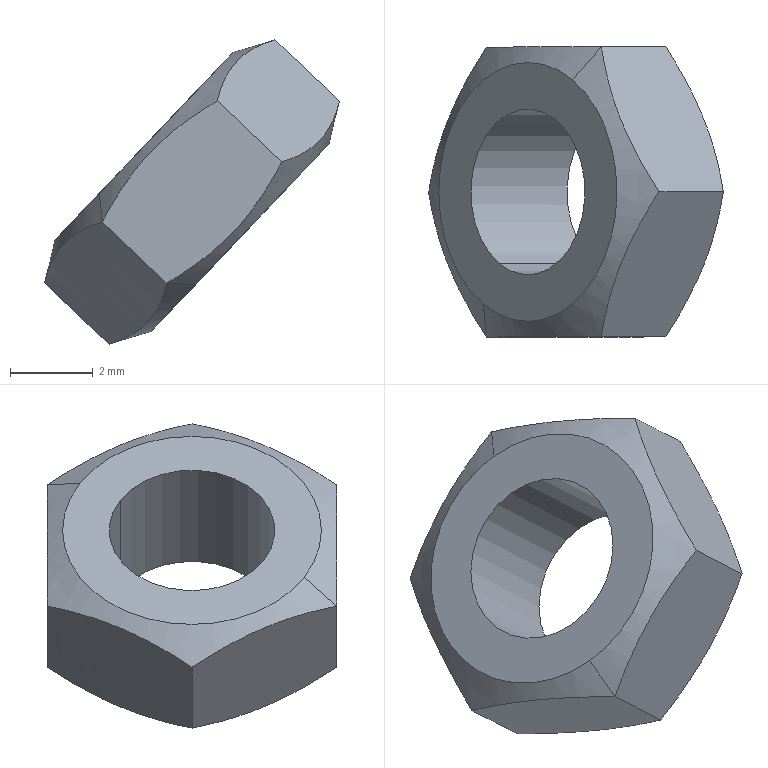Component | SolidWorks | 100-1_hex nuts, style 1-grades ab gb_GB_FASTENER_NUT_SNAB1 M4-N-1 | 1 solid | 14 faces | box 7.11 x 7 x 7.34 mm | volume 91 mm3 | plane 8 | cone 4 | cylinder 2 | commonest cylinder face diameters 4 x2
STEP:
#1=COLOUR_RGB('',0.7922,0.8196,0.9333);
#2=FILL_AREA_STYLE_COLOUR('',#1);
#3=FILL_AREA_STYLE('',(#2));
#4=SURFACE_STYLE_FILL_AREA(#3);
#5=SURFACE_SIDE_STYLE('',(#4));
#6=SURFACE_STYLE_USAGE(.BOTH.,#5);
#7=PRESENTATION_STYLE_ASSIGNMENT((#6));
#8=CARTESIAN_POINT('',(20.163,50.208,-80.248));
#9=VERTEX_POINT('',#8);
#10=CARTESIAN_POINT('',(20.248,50.422,-80.159));
#11=VERTEX_POINT('',#10);
#12=CARTESIAN_POINT('',(20.205,50.315,-80.204));
#13=DIRECTION('',(-0.7258,-0.,0.6879));
#14=DIRECTION('',(0.3439,0.866,0.3629));
#15=AXIS2_PLACEMENT_3D('',#12,#13,#14);
#16=CIRCLE('',#15,0.123);
#17=EDGE_CURVE('',#9,#11,#16,.T.);
#18=ORIENTED_EDGE('',*,*,#17,.T.);
#19=CARTESIAN_POINT('',(20.205,50.315,-80.204));
#20=DIRECTION('',(-0.7258,-0.,0.6879));
#21=DIRECTION('',(0.3439,0.866,0.3629));
#22=AXIS2_PLACEMENT_3D('',#19,#20,#21);
#23=CIRCLE('',#22,0.123);
#24=EDGE_CURVE('',#11,#9,#23,.T.);
#25=ORIENTED_EDGE('',*,*,#24,.T.);
#26=EDGE_LOOP('',(#18,#25));
#27=FACE_OUTER_BOUND('',#26,.T.);
#28=CARTESIAN_POINT('',(20.233,50.383,-80.175));
#29=VERTEX_POINT('',#28);
#30=CARTESIAN_POINT('',(20.178,50.247,-80.232));
#31=VERTEX_POINT('',#30);
#32=CARTESIAN_POINT('',(20.205,50.315,-80.204));
#33=DIRECTION('',(-0.7258,-0.,0.6879));
#34=DIRECTION('',(-0.3439,-0.866,-0.3629));
#35=AXIS2_PLACEMENT_3D('',#32,#33,#34);
#36=CIRCLE('',#35,0.07874);
#37=EDGE_CURVE('',#29,#31,#36,.T.);
#38=ORIENTED_EDGE('',*,*,#37,.F.);
#39=CARTESIAN_POINT('',(20.205,50.315,-80.204));
#40=DIRECTION('',(0.7258,0.,-0.6879));
#41=DIRECTION('',(-0.3439,-0.866,-0.3629));
#42=AXIS2_PLACEMENT_3D('',#39,#40,#41);
#43=CIRCLE('',#42,0.07874);
#44=EDGE_CURVE('',#29,#31,#43,.T.);
#45=ORIENTED_EDGE('',*,*,#44,.T.);
#46=EDGE_LOOP('',(#38,#45));
#47=FACE_BOUND('',#46,.T.);
#48=CARTESIAN_POINT('',(20.151,50.177,-80.262));
#49=DIRECTION('',(0.7258,0.,-0.6879));
#50=DIRECTION('',(-0.3439,-0.866,-0.3629));
#51=AXIS2_PLACEMENT_3D('',#48,#49,#50);
#52=PLANE('',#51);
#53=ADVANCED_FACE('',(#27,#47),#52,.F.);
#54=CARTESIAN_POINT('',(20.255,50.208,-80.335));
#55=VERTEX_POINT('',#54);
#56=CARTESIAN_POINT('',(20.227,50.177,-80.334));
#57=VERTEX_POINT('',#56);
#58=CARTESIAN_POINT('',(20.255,50.208,-80.335));
#59=DIRECTION('',(-0.6608,-0.75,0.02965));
#60=VECTOR('',#59,39.37);
#61=LINE('',#58,#60);
#62=EDGE_CURVE('',#55,#57,#61,.T.);
#63=ORIENTED_EDGE('',*,*,#62,.F.);
#64=CARTESIAN_POINT('',(20.339,50.422,-80.246));
#65=VERTEX_POINT('',#64);
#66=CARTESIAN_POINT('',(20.297,50.315,-80.29));
#67=DIRECTION('',(-0.7258,-0.,0.6879));
#68=DIRECTION('',(0.3439,0.866,0.3629));
#69=AXIS2_PLACEMENT_3D('',#66,#67,#68);
#70=CIRCLE('',#69,0.123);
#71=EDGE_CURVE('',#55,#65,#70,.T.);
#72=ORIENTED_EDGE('',*,*,#71,.T.);
#73=CARTESIAN_POINT('',(20.336,50.453,-80.218));
#74=VERTEX_POINT('',#73);
#75=CARTESIAN_POINT('',(20.339,50.422,-80.246));
#76=DIRECTION('',(-0.06505,0.75,0.6582));
#77=VECTOR('',#76,39.37);
#78=LINE('',#75,#77);
#79=EDGE_CURVE('',#65,#74,#78,.T.);
#80=ORIENTED_EDGE('',*,*,#79,.T.);
#81=CARTESIAN_POINT('',(20.391,50.315,-80.161));
#82=VERTEX_POINT('',#81);
#83=CARTESIAN_POINT('',(20.336,50.453,-80.218));
#84=CARTESIAN_POINT('',(20.34,50.447,-80.217));
#85=CARTESIAN_POINT('',(20.344,50.441,-80.216));
#86=CARTESIAN_POINT('',(20.349,50.433,-80.214));
#87=CARTESIAN_POINT('',(20.35,50.43,-80.213));
#88=CARTESIAN_POINT('',(20.353,50.426,-80.212));
#89=CARTESIAN_POINT('',(20.354,50.424,-80.212));
#90=CARTESIAN_POINT('',(20.355,50.422,-80.211));
#91=CARTESIAN_POINT('',(20.356,50.42,-80.211));
#92=CARTESIAN_POINT('',(20.356,50.419,-80.21));
#93=CARTESIAN_POINT('',(20.36,50.413,-80.209));
#94=CARTESIAN_POINT('',(20.363,50.407,-80.207));
#95=CARTESIAN_POINT('',(20.368,50.396,-80.203));
#96=CARTESIAN_POINT('',(20.37,50.39,-80.2));
#97=CARTESIAN_POINT('',(20.375,50.378,-80.196));
#98=CARTESIAN_POINT('',(20.377,50.372,-80.193));
#99=CARTESIAN_POINT('',(20.38,50.364,-80.189));
#100=CARTESIAN_POINT('',(20.381,50.361,-80.187));
#101=CARTESIAN_POINT('',(20.382,50.356,-80.185));
#102=CARTESIAN_POINT('',(20.383,50.354,-80.184));
#103=CARTESIAN_POINT('',(20.383,50.352,-80.183));
#104=CARTESIAN_POINT('',(20.384,50.351,-80.182));
#105=CARTESIAN_POINT('',(20.384,50.35,-80.181));
#106=CARTESIAN_POINT('',(20.387,50.338,-80.175));
#107=CARTESIAN_POINT('',(20.389,50.327,-80.168));
#108=CARTESIAN_POINT('',(20.391,50.315,-80.161));
#109=B_SPLINE_CURVE_WITH_KNOTS('',3,(#83,#84,#85,#86,#87,#88,#89,#90,#91,#92,#93,#94,#95,#96,#97,#98,#99,#100,#101,#102,#103,#104,#105,#106,#107,#108),.UNSPECIFIED.,.F.,.F.,(4,2,2,1,2,2,2,2,2,2,1,2,2,4),(0.,0.125,0.1875,0.2187,0.2344,0.25,0.375,0.5,0.625,0.6875,0.7188,0.7344,0.75,1.),.UNSPECIFIED.);
#110=EDGE_CURVE('',#74,#82,#109,.T.);
#111=ORIENTED_EDGE('',*,*,#110,.T.);
#112=CARTESIAN_POINT('',(20.336,50.177,-80.218));
#113=VERTEX_POINT('',#112);
#114=CARTESIAN_POINT('',(20.391,50.315,-80.161));
#115=CARTESIAN_POINT('',(20.39,50.309,-80.164));
#116=CARTESIAN_POINT('',(20.389,50.303,-80.168));
#117=CARTESIAN_POINT('',(20.388,50.295,-80.173));
#118=CARTESIAN_POINT('',(20.387,50.292,-80.175));
#119=CARTESIAN_POINT('',(20.386,50.288,-80.177));
#120=CARTESIAN_POINT('',(20.385,50.286,-80.178));
#121=CARTESIAN_POINT('',(20.385,50.284,-80.18));
#122=CARTESIAN_POINT('',(20.385,50.282,-80.18));
#123=CARTESIAN_POINT('',(20.384,50.282,-80.181));
#124=CARTESIAN_POINT('',(20.381,50.269,-80.188));
#125=CARTESIAN_POINT('',(20.377,50.258,-80.193));
#126=CARTESIAN_POINT('',(20.372,50.243,-80.199));
#127=CARTESIAN_POINT('',(20.37,50.24,-80.2));
#128=CARTESIAN_POINT('',(20.368,50.234,-80.203));
#129=CARTESIAN_POINT('',(20.367,50.231,-80.204));
#130=CARTESIAN_POINT('',(20.364,50.226,-80.206));
#131=CARTESIAN_POINT('',(20.362,50.223,-80.207));
#132=CARTESIAN_POINT('',(20.36,50.218,-80.208));
#133=CARTESIAN_POINT('',(20.36,50.217,-80.209));
#134=CARTESIAN_POINT('',(20.358,50.214,-80.209));
#135=CARTESIAN_POINT('',(20.357,50.212,-80.21));
#136=CARTESIAN_POINT('',(20.351,50.2,-80.214));
#137=CARTESIAN_POINT('',(20.344,50.189,-80.216));
#138=CARTESIAN_POINT('',(20.336,50.177,-80.218));
#139=B_SPLINE_CURVE_WITH_KNOTS('',3,(#114,#115,#116,#117,#118,#119,#120,#121,#122,#123,#124,#125,#126,#127,#128,#129,#130,#131,#132,#133,#134,#135,#136,#137,#138),.UNSPECIFIED.,.F.,.F.,(4,2,2,1,2,2,2,2,2,2,2,2,4),(0.,0.125,0.1875,0.2188,0.2344,0.25,0.5,0.5625,0.625,0.6875,0.7188,0.75,1.),.UNSPECIFIED.);
#140=EDGE_CURVE('',#82,#113,#139,.T.);
#141=ORIENTED_EDGE('',*,*,#140,.T.);
#142=CARTESIAN_POINT('',(20.336,50.177,-80.218));
#143=CARTESIAN_POINT('',(20.333,50.177,-80.225));
#144=CARTESIAN_POINT('',(20.33,50.177,-80.231));
#145=CARTESIAN_POINT('',(20.325,50.177,-80.239));
#146=CARTESIAN_POINT('',(20.323,50.177,-80.242));
#147=CARTESIAN_POINT('',(20.32,50.177,-80.246));
#148=CARTESIAN_POINT('',(20.319,50.177,-80.248));
#149=CARTESIAN_POINT('',(20.318,50.177,-80.25));
#150=CARTESIAN_POINT('',(20.317,50.177,-80.252));
#151=CARTESIAN_POINT('',(20.316,50.177,-80.252));
#152=CARTESIAN_POINT('',(20.312,50.177,-80.259));
#153=CARTESIAN_POINT('',(20.308,50.177,-80.264));
#154=CARTESIAN_POINT('',(20.3,50.177,-80.275));
#155=CARTESIAN_POINT('',(20.295,50.177,-80.28));
#156=CARTESIAN_POINT('',(20.286,50.177,-80.289));
#157=CARTESIAN_POINT('',(20.281,50.177,-80.294));
#158=CARTESIAN_POINT('',(20.274,50.177,-80.301));
#159=CARTESIAN_POINT('',(20.271,50.177,-80.303));
#160=CARTESIAN_POINT('',(20.267,50.177,-80.306));
#161=CARTESIAN_POINT('',(20.265,50.177,-80.308));
#162=CARTESIAN_POINT('',(20.263,50.177,-80.309));
#163=CARTESIAN_POINT('',(20.262,50.177,-80.31));
#164=CARTESIAN_POINT('',(20.261,50.177,-80.311));
#165=CARTESIAN_POINT('',(20.25,50.177,-80.319));
#166=CARTESIAN_POINT('',(20.239,50.177,-80.327));
#167=CARTESIAN_POINT('',(20.227,50.177,-80.334));
#168=B_SPLINE_CURVE_WITH_KNOTS('',3,(#142,#143,#144,#145,#146,#147,#148,#149,#150,#151,#152,#153,#154,#155,#156,#157,#158,#159,#160,#161,#162,#163,#164,#165,#166,#167),.UNSPECIFIED.,.F.,.F.,(4,2,2,1,2,2,2,2,2,2,1,2,2,4),(0.,0.125,0.1875,0.2188,0.2344,0.25,0.375,0.5,0.625,0.6875,0.7188,0.7344,0.75,1.),.UNSPECIFIED.);
#169=EDGE_CURVE('',#113,#57,#168,.T.);
#170=ORIENTED_EDGE('',*,*,#169,.T.);
#171=EDGE_LOOP('',(#63,#72,#80,#111,#141,#170));
#172=FACE_OUTER_BOUND('',#171,.T.);
#173=CARTESIAN_POINT('',(20.297,50.315,-80.29));
#174=DIRECTION('',(-0.7258,-0.,0.6879));
#175=DIRECTION('',(0.3439,0.866,0.3629));
#176=AXIS2_PLACEMENT_3D('',#173,#174,#175);
#177=CONICAL_SURFACE('',#176,0.123,1.047);
#178=ADVANCED_FACE('',(#172),#177,.T.);
#179=CARTESIAN_POINT('',(20.275,50.453,-80.16));
#180=VERTEX_POINT('',#179);
#181=CARTESIAN_POINT('',(20.275,50.453,-80.16));
#182=DIRECTION('',(0.6608,0.75,-0.02965));
#183=VECTOR('',#182,39.37);
#184=LINE('',#181,#183);
#185=EDGE_CURVE('',#11,#180,#184,.T.);
#186=ORIENTED_EDGE('',*,*,#185,.F.);
#187=ORIENTED_EDGE('',*,*,#17,.F.);
#188=CARTESIAN_POINT('',(20.166,50.177,-80.276));
#189=VERTEX_POINT('',#188);
#190=CARTESIAN_POINT('',(20.166,50.177,-80.276));
#191=DIRECTION('',(0.06505,-0.75,-0.6582));
#192=VECTOR('',#191,39.37);
#193=LINE('',#190,#192);
#194=EDGE_CURVE('',#9,#189,#193,.T.);
#195=ORIENTED_EDGE('',*,*,#194,.T.);
#196=CARTESIAN_POINT('',(20.275,50.177,-80.16));
#197=VERTEX_POINT('',#196);
#198=CARTESIAN_POINT('',(20.166,50.177,-80.276));
#199=CARTESIAN_POINT('',(20.169,50.177,-80.27));
#200=CARTESIAN_POINT('',(20.172,50.177,-80.264));
#201=CARTESIAN_POINT('',(20.177,50.177,-80.255));
#202=CARTESIAN_POINT('',(20.179,50.177,-80.252));
#203=CARTESIAN_POINT('',(20.182,50.177,-80.248));
#204=CARTESIAN_POINT('',(20.183,50.177,-80.246));
#205=CARTESIAN_POINT('',(20.185,50.177,-80.244));
#206=CARTESIAN_POINT('',(20.185,50.177,-80.242));
#207=CARTESIAN_POINT('',(20.186,50.177,-80.242));
#208=CARTESIAN_POINT('',(20.19,50.177,-80.235));
#209=CARTESIAN_POINT('',(20.194,50.177,-80.23));
#210=CARTESIAN_POINT('',(20.203,50.177,-80.22));
#211=CARTESIAN_POINT('',(20.207,50.177,-80.215));
#212=CARTESIAN_POINT('',(20.216,50.177,-80.205));
#213=CARTESIAN_POINT('',(20.221,50.177,-80.2));
#214=CARTESIAN_POINT('',(20.228,50.177,-80.194));
#215=CARTESIAN_POINT('',(20.231,50.177,-80.191));
#216=CARTESIAN_POINT('',(20.235,50.177,-80.188));
#217=CARTESIAN_POINT('',(20.237,50.177,-80.186));
#218=CARTESIAN_POINT('',(20.239,50.177,-80.185));
#219=CARTESIAN_POINT('',(20.24,50.177,-80.184));
#220=CARTESIAN_POINT('',(20.241,50.177,-80.183));
#221=CARTESIAN_POINT('',(20.252,50.177,-80.175));
#222=CARTESIAN_POINT('',(20.263,50.177,-80.168));
#223=CARTESIAN_POINT('',(20.275,50.177,-80.16));
#224=B_SPLINE_CURVE_WITH_KNOTS('',3,(#198,#199,#200,#201,#202,#203,#204,#205,#206,#207,#208,#209,#210,#211,#212,#213,#214,#215,#216,#217,#218,#219,#220,#221,#222,#223),.UNSPECIFIED.,.F.,.F.,(4,2,2,1,2,2,2,2,2,2,1,2,2,4),(0.,0.125,0.1875,0.2188,0.2344,0.25,0.375,0.5,0.625,0.6875,0.7188,0.7344,0.75,1.),.UNSPECIFIED.);
#225=EDGE_CURVE('',#189,#197,#224,.T.);
#226=ORIENTED_EDGE('',*,*,#225,.T.);
#227=CARTESIAN_POINT('',(20.33,50.315,-80.103));
#228=VERTEX_POINT('',#227);
#229=CARTESIAN_POINT('',(20.275,50.177,-80.16));
#230=CARTESIAN_POINT('',(20.276,50.183,-80.157));
#231=CARTESIAN_POINT('',(20.277,50.189,-80.153));
#232=CARTESIAN_POINT('',(20.279,50.197,-80.148));
#233=CARTESIAN_POINT('',(20.28,50.2,-80.146));
#234=CARTESIAN_POINT('',(20.281,50.204,-80.144));
#235=CARTESIAN_POINT('',(20.281,50.206,-80.143));
#236=CARTESIAN_POINT('',(20.282,50.208,-80.142));
#237=CARTESIAN_POINT('',(20.282,50.21,-80.141));
#238=CARTESIAN_POINT('',(20.283,50.214,-80.138));
#239=CARTESIAN_POINT('',(20.284,50.217,-80.137));
#240=CARTESIAN_POINT('',(20.286,50.223,-80.134));
#241=CARTESIAN_POINT('',(20.286,50.226,-80.132));
#242=CARTESIAN_POINT('',(20.289,50.234,-80.128));
#243=CARTESIAN_POINT('',(20.291,50.24,-80.125));
#244=CARTESIAN_POINT('',(20.296,50.252,-80.121));
#245=CARTESIAN_POINT('',(20.298,50.258,-80.118));
#246=CARTESIAN_POINT('',(20.302,50.266,-80.115));
#247=CARTESIAN_POINT('',(20.304,50.269,-80.114));
#248=CARTESIAN_POINT('',(20.306,50.273,-80.113));
#249=CARTESIAN_POINT('',(20.307,50.276,-80.112));
#250=CARTESIAN_POINT('',(20.308,50.278,-80.112));
#251=CARTESIAN_POINT('',(20.309,50.279,-80.111));
#252=CARTESIAN_POINT('',(20.31,50.28,-80.111));
#253=CARTESIAN_POINT('',(20.316,50.292,-80.107));
#254=CARTESIAN_POINT('',(20.322,50.303,-80.105));
#255=CARTESIAN_POINT('',(20.33,50.315,-80.103));
#256=B_SPLINE_CURVE_WITH_KNOTS('',3,(#229,#230,#231,#232,#233,#234,#235,#236,#237,#238,#239,#240,#241,#242,#243,#244,#245,#246,#247,#248,#249,#250,#251,#252,#253,#254,#255),.UNSPECIFIED.,.F.,.F.,(4,2,2,2,2,2,2,2,2,2,1,2,2,4),(0.,0.125,0.1875,0.2188,0.25,0.3125,0.375,0.5,0.625,0.6875,0.7188,0.7344,0.75,1.),.UNSPECIFIED.);
#257=EDGE_CURVE('',#197,#228,#256,.T.);
#258=ORIENTED_EDGE('',*,*,#257,.T.);
#259=CARTESIAN_POINT('',(20.33,50.315,-80.103));
#260=CARTESIAN_POINT('',(20.326,50.321,-80.104));
#261=CARTESIAN_POINT('',(20.323,50.327,-80.105));
#262=CARTESIAN_POINT('',(20.318,50.335,-80.107));
#263=CARTESIAN_POINT('',(20.316,50.338,-80.108));
#264=CARTESIAN_POINT('',(20.314,50.342,-80.109));
#265=CARTESIAN_POINT('',(20.313,50.344,-80.109));
#266=CARTESIAN_POINT('',(20.311,50.346,-80.11));
#267=CARTESIAN_POINT('',(20.311,50.348,-80.11));
#268=CARTESIAN_POINT('',(20.31,50.348,-80.11));
#269=CARTESIAN_POINT('',(20.307,50.355,-80.112));
#270=CARTESIAN_POINT('',(20.304,50.361,-80.114));
#271=CARTESIAN_POINT('',(20.299,50.372,-80.118));
#272=CARTESIAN_POINT('',(20.296,50.378,-80.121));
#273=CARTESIAN_POINT('',(20.291,50.39,-80.125));
#274=CARTESIAN_POINT('',(20.289,50.395,-80.128));
#275=CARTESIAN_POINT('',(20.286,50.404,-80.132));
#276=CARTESIAN_POINT('',(20.286,50.407,-80.134));
#277=CARTESIAN_POINT('',(20.284,50.411,-80.136));
#278=CARTESIAN_POINT('',(20.284,50.413,-80.137));
#279=CARTESIAN_POINT('',(20.283,50.416,-80.138));
#280=CARTESIAN_POINT('',(20.283,50.417,-80.139));
#281=CARTESIAN_POINT('',(20.282,50.418,-80.139));
#282=CARTESIAN_POINT('',(20.279,50.43,-80.146));
#283=CARTESIAN_POINT('',(20.277,50.441,-80.153));
#284=CARTESIAN_POINT('',(20.275,50.453,-80.16));
#285=B_SPLINE_CURVE_WITH_KNOTS('',3,(#259,#260,#261,#262,#263,#264,#265,#266,#267,#268,#269,#270,#271,#272,#273,#274,#275,#276,#277,#278,#279,#280,#281,#282,#283,#284),.UNSPECIFIED.,.F.,.F.,(4,2,2,1,2,2,2,2,2,2,1,2,2,4),(0.,0.125,0.1875,0.2188,0.2344,0.25,0.375,0.5,0.625,0.6875,0.7187,0.7344,0.75,1.),.UNSPECIFIED.);
#286=EDGE_CURVE('',#228,#180,#285,.T.);
#287=ORIENTED_EDGE('',*,*,#286,.T.);
#288=EDGE_LOOP('',(#186,#187,#195,#226,#258,#287));
#289=FACE_OUTER_BOUND('',#288,.T.);
#290=CARTESIAN_POINT('',(20.221,50.315,-80.218));
#291=DIRECTION('',(0.7258,0.,-0.6879));
#292=DIRECTION('',(-0.3439,-0.866,-0.3629));
#293=AXIS2_PLACEMENT_3D('',#290,#291,#292);
#294=CONICAL_SURFACE('',#293,0.1591,1.047);
#295=ADVANCED_FACE('',(#289),#294,.T.);
#296=CARTESIAN_POINT('',(20.324,50.383,-80.262));
#297=VERTEX_POINT('',#296);
#298=CARTESIAN_POINT('',(20.233,50.383,-80.175));
#299=DIRECTION('',(0.7258,0.,-0.6879));
#300=VECTOR('',#299,39.37);
#301=LINE('',#298,#300);
#302=EDGE_CURVE('',#29,#297,#301,.T.);
#303=ORIENTED_EDGE('',*,*,#302,.F.);
#304=ORIENTED_EDGE('',*,*,#37,.T.);
#305=CARTESIAN_POINT('',(20.27,50.247,-80.319));
#306=VERTEX_POINT('',#305);
#307=CARTESIAN_POINT('',(20.178,50.247,-80.232));
#308=DIRECTION('',(0.7258,0.,-0.6879));
#309=VECTOR('',#308,39.37);
#310=LINE('',#307,#309);
#311=EDGE_CURVE('',#31,#306,#310,.T.);
#312=ORIENTED_EDGE('',*,*,#311,.T.);
#313=CARTESIAN_POINT('',(20.297,50.315,-80.29));
#314=DIRECTION('',(0.7258,0.,-0.6879));
#315=DIRECTION('',(-0.3439,-0.866,-0.3629));
#316=AXIS2_PLACEMENT_3D('',#313,#314,#315);
#317=CIRCLE('',#316,0.07874);
#318=EDGE_CURVE('',#306,#297,#317,.T.);
#319=ORIENTED_EDGE('',*,*,#318,.T.);
#320=EDGE_LOOP('',(#303,#304,#312,#319));
#321=FACE_OUTER_BOUND('',#320,.T.);
#322=CARTESIAN_POINT('',(20.205,50.315,-80.204));
#323=DIRECTION('',(0.7258,0.,-0.6879));
#324=DIRECTION('',(-0.3439,-0.866,-0.3629));
#325=AXIS2_PLACEMENT_3D('',#322,#323,#324);
#326=CYLINDRICAL_SURFACE('',#325,0.07874);
#327=ADVANCED_FACE('',(#321),#326,.F.);
#328=CARTESIAN_POINT('',(20.297,50.315,-80.29));
#329=DIRECTION('',(-0.7258,-0.,0.6879));
#330=DIRECTION('',(-0.3439,-0.866,-0.3629));
#331=AXIS2_PLACEMENT_3D('',#328,#329,#330);
#332=CIRCLE('',#331,0.07874);
#333=EDGE_CURVE('',#306,#297,#332,.T.);
#334=ORIENTED_EDGE('',*,*,#333,.T.);
#335=ORIENTED_EDGE('',*,*,#318,.F.);
#336=EDGE_LOOP('',(#334,#335));
#337=FACE_BOUND('',#336,.T.);
#338=CARTESIAN_POINT('',(20.297,50.315,-80.29));
#339=DIRECTION('',(-0.7258,-0.,0.6879));
#340=DIRECTION('',(0.3439,0.866,0.3629));
#341=AXIS2_PLACEMENT_3D('',#338,#339,#340);
#342=CIRCLE('',#341,0.123);
#343=EDGE_CURVE('',#65,#55,#342,.T.);
#344=ORIENTED_EDGE('',*,*,#343,.F.);
#345=ORIENTED_EDGE('',*,*,#71,.F.);
#346=EDGE_LOOP('',(#344,#345));
#347=FACE_OUTER_BOUND('',#346,.T.);
#348=CARTESIAN_POINT('',(20.242,50.177,-80.348));
#349=DIRECTION('',(0.7258,0.,-0.6879));
#350=DIRECTION('',(-0.3439,-0.866,-0.3629));
#351=AXIS2_PLACEMENT_3D('',#348,#349,#350);
#352=PLANE('',#351);
#353=ADVANCED_FACE('',(#337,#347),#352,.T.);
#354=CARTESIAN_POINT('',(20.172,50.315,-80.392));
#355=VERTEX_POINT('',#354);
#356=CARTESIAN_POINT('',(20.227,50.177,-80.334));
#357=CARTESIAN_POINT('',(20.226,50.183,-80.338));
#358=CARTESIAN_POINT('',(20.225,50.189,-80.341));
#359=CARTESIAN_POINT('',(20.223,50.197,-80.346));
#360=CARTESIAN_POINT('',(20.223,50.2,-80.348));
#361=CARTESIAN_POINT('',(20.222,50.204,-80.35));
#362=CARTESIAN_POINT('',(20.221,50.206,-80.352));
#363=CARTESIAN_POINT('',(20.221,50.208,-80.353));
#364=CARTESIAN_POINT('',(20.22,50.21,-80.354));
#365=CARTESIAN_POINT('',(20.22,50.21,-80.354));
#366=CARTESIAN_POINT('',(20.218,50.217,-80.358));
#367=CARTESIAN_POINT('',(20.217,50.223,-80.361));
#368=CARTESIAN_POINT('',(20.213,50.234,-80.366));
#369=CARTESIAN_POINT('',(20.211,50.24,-80.369));
#370=CARTESIAN_POINT('',(20.206,50.252,-80.374));
#371=CARTESIAN_POINT('',(20.204,50.258,-80.376));
#372=CARTESIAN_POINT('',(20.2,50.266,-80.379));
#373=CARTESIAN_POINT('',(20.198,50.269,-80.38));
#374=CARTESIAN_POINT('',(20.196,50.273,-80.381));
#375=CARTESIAN_POINT('',(20.195,50.276,-80.382));
#376=CARTESIAN_POINT('',(20.194,50.278,-80.383));
#377=CARTESIAN_POINT('',(20.193,50.279,-80.383));
#378=CARTESIAN_POINT('',(20.193,50.28,-80.383));
#379=CARTESIAN_POINT('',(20.186,50.292,-80.387));
#380=CARTESIAN_POINT('',(20.18,50.303,-80.389));
#381=CARTESIAN_POINT('',(20.172,50.315,-80.392));
#382=B_SPLINE_CURVE_WITH_KNOTS('',3,(#356,#357,#358,#359,#360,#361,#362,#363,#364,#365,#366,#367,#368,#369,#370,#371,#372,#373,#374,#375,#376,#377,#378,#379,#380,#381),.UNSPECIFIED.,.F.,.F.,(4,2,2,1,2,2,2,2,2,2,1,2,2,4),(0.,0.125,0.1875,0.2187,0.2344,0.25,0.375,0.5,0.625,0.6875,0.7187,0.7344,0.75,1.),.UNSPECIFIED.);
#383=EDGE_CURVE('',#57,#355,#382,.T.);
#384=ORIENTED_EDGE('',*,*,#383,.F.);
#385=CARTESIAN_POINT('',(20.151,50.177,-80.262));
#386=DIRECTION('',(0.7258,0.,-0.6879));
#387=VECTOR('',#386,39.37);
#388=LINE('',#385,#387);
#389=EDGE_CURVE('',#189,#57,#388,.T.);
#390=ORIENTED_EDGE('',*,*,#389,.F.);
#391=CARTESIAN_POINT('',(20.111,50.315,-80.334));
#392=VERTEX_POINT('',#391);
#393=CARTESIAN_POINT('',(20.111,50.315,-80.334));
#394=CARTESIAN_POINT('',(20.112,50.309,-80.33));
#395=CARTESIAN_POINT('',(20.113,50.303,-80.326));
#396=CARTESIAN_POINT('',(20.115,50.295,-80.321));
#397=CARTESIAN_POINT('',(20.115,50.292,-80.319));
#398=CARTESIAN_POINT('',(20.116,50.288,-80.317));
#399=CARTESIAN_POINT('',(20.117,50.286,-80.316));
#400=CARTESIAN_POINT('',(20.117,50.284,-80.315));
#401=CARTESIAN_POINT('',(20.118,50.282,-80.314));
#402=CARTESIAN_POINT('',(20.118,50.282,-80.314));
#403=CARTESIAN_POINT('',(20.12,50.275,-80.31));
#404=CARTESIAN_POINT('',(20.121,50.269,-80.307));
#405=CARTESIAN_POINT('',(20.125,50.258,-80.301));
#406=CARTESIAN_POINT('',(20.127,50.252,-80.299));
#407=CARTESIAN_POINT('',(20.132,50.24,-80.294));
#408=CARTESIAN_POINT('',(20.134,50.235,-80.292));
#409=CARTESIAN_POINT('',(20.138,50.226,-80.289));
#410=CARTESIAN_POINT('',(20.14,50.223,-80.288));
#411=CARTESIAN_POINT('',(20.142,50.219,-80.286));
#412=CARTESIAN_POINT('',(20.143,50.216,-80.285));
#413=CARTESIAN_POINT('',(20.144,50.214,-80.285));
#414=CARTESIAN_POINT('',(20.145,50.213,-80.284));
#415=CARTESIAN_POINT('',(20.145,50.212,-80.284));
#416=CARTESIAN_POINT('',(20.152,50.2,-80.281));
#417=CARTESIAN_POINT('',(20.158,50.189,-80.278));
#418=CARTESIAN_POINT('',(20.166,50.177,-80.276));
#419=B_SPLINE_CURVE_WITH_KNOTS('',3,(#393,#394,#395,#396,#397,#398,#399,#400,#401,#402,#403,#404,#405,#406,#407,#408,#409,#410,#411,#412,#413,#414,#415,#416,#417,#418),.UNSPECIFIED.,.F.,.F.,(4,2,2,1,2,2,2,2,2,2,1,2,2,4),(0.,0.125,0.1875,0.2187,0.2344,0.25,0.375,0.5,0.625,0.6875,0.7187,0.7344,0.75,1.),.UNSPECIFIED.);
#420=EDGE_CURVE('',#392,#189,#419,.T.);
#421=ORIENTED_EDGE('',*,*,#420,.F.);
#422=CARTESIAN_POINT('',(20.096,50.315,-80.319));
#423=DIRECTION('',(0.7258,0.,-0.6879));
#424=VECTOR('',#423,39.37);
#425=LINE('',#422,#424);
#426=EDGE_CURVE('',#392,#355,#425,.T.);
#427=ORIENTED_EDGE('',*,*,#426,.T.);
#428=EDGE_LOOP('',(#384,#390,#421,#427));
#429=FACE_OUTER_BOUND('',#428,.T.);
#430=CARTESIAN_POINT('',(20.151,50.177,-80.262));
#431=DIRECTION('',(-0.5957,-0.5,-0.6286));
#432=DIRECTION('',(-0.7258,-0.,0.6879));
#433=AXIS2_PLACEMENT_3D('',#430,#431,#432);
#434=PLANE('',#433);
#435=ADVANCED_FACE('',(#429),#434,.T.);
#436=CARTESIAN_POINT('',(20.227,50.453,-80.334));
#437=VERTEX_POINT('',#436);
#438=CARTESIAN_POINT('',(20.172,50.315,-80.392));
#439=CARTESIAN_POINT('',(20.176,50.321,-80.39));
#440=CARTESIAN_POINT('',(20.18,50.327,-80.389));
#441=CARTESIAN_POINT('',(20.185,50.335,-80.387));
#442=CARTESIAN_POINT('',(20.186,50.338,-80.387));
#443=CARTESIAN_POINT('',(20.189,50.342,-80.385));
#444=CARTESIAN_POINT('',(20.189,50.343,-80.385));
#445=CARTESIAN_POINT('',(20.191,50.346,-80.384));
#446=CARTESIAN_POINT('',(20.192,50.347,-80.384));
#447=CARTESIAN_POINT('',(20.194,50.352,-80.383));
#448=CARTESIAN_POINT('',(20.195,50.355,-80.382));
#449=CARTESIAN_POINT('',(20.198,50.361,-80.38));
#450=CARTESIAN_POINT('',(20.2,50.363,-80.379));
#451=CARTESIAN_POINT('',(20.204,50.372,-80.376));
#452=CARTESIAN_POINT('',(20.206,50.378,-80.374));
#453=CARTESIAN_POINT('',(20.211,50.39,-80.369));
#454=CARTESIAN_POINT('',(20.213,50.395,-80.366));
#455=CARTESIAN_POINT('',(20.216,50.404,-80.362));
#456=CARTESIAN_POINT('',(20.217,50.407,-80.361));
#457=CARTESIAN_POINT('',(20.218,50.411,-80.358));
#458=CARTESIAN_POINT('',(20.219,50.413,-80.357));
#459=CARTESIAN_POINT('',(20.219,50.416,-80.356));
#460=CARTESIAN_POINT('',(20.22,50.417,-80.355));
#461=CARTESIAN_POINT('',(20.22,50.418,-80.355));
#462=CARTESIAN_POINT('',(20.223,50.43,-80.348));
#463=CARTESIAN_POINT('',(20.225,50.441,-80.341));
#464=CARTESIAN_POINT('',(20.227,50.453,-80.334));
#465=B_SPLINE_CURVE_WITH_KNOTS('',3,(#438,#439,#440,#441,#442,#443,#444,#445,#446,#447,#448,#449,#450,#451,#452,#453,#454,#455,#456,#457,#458,#459,#460,#461,#462,#463,#464),.UNSPECIFIED.,.F.,.F.,(4,2,2,2,2,2,2,2,2,2,1,2,2,4),(0.,0.125,0.1875,0.2188,0.25,0.3125,0.375,0.5,0.625,0.6875,0.7188,0.7344,0.75,1.),.UNSPECIFIED.);
#466=EDGE_CURVE('',#355,#437,#465,.T.);
#467=ORIENTED_EDGE('',*,*,#466,.F.);
#468=ORIENTED_EDGE('',*,*,#426,.F.);
#469=CARTESIAN_POINT('',(20.166,50.453,-80.276));
#470=VERTEX_POINT('',#469);
#471=CARTESIAN_POINT('',(20.166,50.453,-80.276));
#472=CARTESIAN_POINT('',(20.162,50.447,-80.277));
#473=CARTESIAN_POINT('',(20.159,50.441,-80.278));
#474=CARTESIAN_POINT('',(20.154,50.433,-80.28));
#475=CARTESIAN_POINT('',(20.152,50.43,-80.281));
#476=CARTESIAN_POINT('',(20.15,50.426,-80.282));
#477=CARTESIAN_POINT('',(20.148,50.423,-80.283));
#478=CARTESIAN_POINT('',(20.147,50.421,-80.283));
#479=CARTESIAN_POINT('',(20.146,50.42,-80.284));
#480=CARTESIAN_POINT('',(20.146,50.419,-80.284));
#481=CARTESIAN_POINT('',(20.139,50.407,-80.287));
#482=CARTESIAN_POINT('',(20.134,50.396,-80.291));
#483=CARTESIAN_POINT('',(20.128,50.381,-80.297));
#484=CARTESIAN_POINT('',(20.127,50.378,-80.299));
#485=CARTESIAN_POINT('',(20.125,50.372,-80.301));
#486=CARTESIAN_POINT('',(20.124,50.369,-80.303));
#487=CARTESIAN_POINT('',(20.122,50.363,-80.306));
#488=CARTESIAN_POINT('',(20.121,50.361,-80.307));
#489=CARTESIAN_POINT('',(20.12,50.356,-80.309));
#490=CARTESIAN_POINT('',(20.12,50.355,-80.31));
#491=CARTESIAN_POINT('',(20.119,50.352,-80.312));
#492=CARTESIAN_POINT('',(20.118,50.35,-80.312));
#493=CARTESIAN_POINT('',(20.115,50.338,-80.319));
#494=CARTESIAN_POINT('',(20.113,50.327,-80.326));
#495=CARTESIAN_POINT('',(20.111,50.315,-80.334));
#496=B_SPLINE_CURVE_WITH_KNOTS('',3,(#471,#472,#473,#474,#475,#476,#477,#478,#479,#480,#481,#482,#483,#484,#485,#486,#487,#488,#489,#490,#491,#492,#493,#494,#495),.UNSPECIFIED.,.F.,.F.,(4,2,2,1,2,2,2,2,2,2,2,2,4),(0.,0.125,0.1875,0.2187,0.2344,0.25,0.5,0.5625,0.625,0.6875,0.7187,0.75,1.),.UNSPECIFIED.);
#497=EDGE_CURVE('',#470,#392,#496,.T.);
#498=ORIENTED_EDGE('',*,*,#497,.F.);
#499=CARTESIAN_POINT('',(20.151,50.453,-80.262));
#500=DIRECTION('',(0.7258,0.,-0.6879));
#501=VECTOR('',#500,39.37);
#502=LINE('',#499,#501);
#503=EDGE_CURVE('',#470,#437,#502,.T.);
#504=ORIENTED_EDGE('',*,*,#503,.T.);
#505=EDGE_LOOP('',(#467,#468,#498,#504));
#506=FACE_OUTER_BOUND('',#505,.T.);
#507=CARTESIAN_POINT('',(20.096,50.315,-80.319));
#508=DIRECTION('',(-0.5957,0.5,-0.6286));
#509=DIRECTION('',(-0.3439,-0.866,-0.3629));
#510=AXIS2_PLACEMENT_3D('',#507,#508,#509);
#511=PLANE('',#510);
#512=ADVANCED_FACE('',(#506),#511,.T.);
#513=CARTESIAN_POINT('',(20.227,50.453,-80.334));
#514=CARTESIAN_POINT('',(20.233,50.453,-80.33));
#515=CARTESIAN_POINT('',(20.239,50.453,-80.327));
#516=CARTESIAN_POINT('',(20.247,50.453,-80.321));
#517=CARTESIAN_POINT('',(20.25,50.453,-80.319));
#518=CARTESIAN_POINT('',(20.254,50.453,-80.316));
#519=CARTESIAN_POINT('',(20.256,50.453,-80.315));
#520=CARTESIAN_POINT('',(20.258,50.453,-80.313));
#521=CARTESIAN_POINT('',(20.259,50.453,-80.312));
#522=CARTESIAN_POINT('',(20.26,50.453,-80.312));
#523=CARTESIAN_POINT('',(20.266,50.453,-80.307));
#524=CARTESIAN_POINT('',(20.271,50.453,-80.303));
#525=CARTESIAN_POINT('',(20.281,50.453,-80.294));
#526=CARTESIAN_POINT('',(20.286,50.453,-80.29));
#527=CARTESIAN_POINT('',(20.295,50.453,-80.28));
#528=CARTESIAN_POINT('',(20.3,50.453,-80.275));
#529=CARTESIAN_POINT('',(20.306,50.453,-80.267));
#530=CARTESIAN_POINT('',(20.308,50.453,-80.264));
#531=CARTESIAN_POINT('',(20.311,50.453,-80.26));
#532=CARTESIAN_POINT('',(20.312,50.453,-80.258));
#533=CARTESIAN_POINT('',(20.314,50.453,-80.256));
#534=CARTESIAN_POINT('',(20.315,50.453,-80.255));
#535=CARTESIAN_POINT('',(20.315,50.453,-80.254));
#536=CARTESIAN_POINT('',(20.323,50.453,-80.242));
#537=CARTESIAN_POINT('',(20.33,50.453,-80.231));
#538=CARTESIAN_POINT('',(20.336,50.453,-80.218));
#539=B_SPLINE_CURVE_WITH_KNOTS('',3,(#513,#514,#515,#516,#517,#518,#519,#520,#521,#522,#523,#524,#525,#526,#527,#528,#529,#530,#531,#532,#533,#534,#535,#536,#537,#538),.UNSPECIFIED.,.F.,.F.,(4,2,2,1,2,2,2,2,2,2,1,2,2,4),(0.,0.125,0.1875,0.2188,0.2344,0.25,0.375,0.5,0.625,0.6875,0.7188,0.7344,0.75,1.),.UNSPECIFIED.);
#540=EDGE_CURVE('',#437,#74,#539,.T.);
#541=ORIENTED_EDGE('',*,*,#540,.F.);
#542=ORIENTED_EDGE('',*,*,#503,.F.);
#543=CARTESIAN_POINT('',(20.275,50.453,-80.16));
#544=CARTESIAN_POINT('',(20.269,50.453,-80.164));
#545=CARTESIAN_POINT('',(20.263,50.453,-80.168));
#546=CARTESIAN_POINT('',(20.255,50.453,-80.173));
#547=CARTESIAN_POINT('',(20.252,50.453,-80.175));
#548=CARTESIAN_POINT('',(20.248,50.453,-80.178));
#549=CARTESIAN_POINT('',(20.246,50.453,-80.179));
#550=CARTESIAN_POINT('',(20.244,50.453,-80.181));
#551=CARTESIAN_POINT('',(20.243,50.453,-80.182));
#552=CARTESIAN_POINT('',(20.242,50.453,-80.182));
#553=CARTESIAN_POINT('',(20.236,50.453,-80.187));
#554=CARTESIAN_POINT('',(20.231,50.453,-80.191));
#555=CARTESIAN_POINT('',(20.221,50.453,-80.2));
#556=CARTESIAN_POINT('',(20.216,50.453,-80.205));
#557=CARTESIAN_POINT('',(20.207,50.453,-80.214));
#558=CARTESIAN_POINT('',(20.203,50.453,-80.219));
#559=CARTESIAN_POINT('',(20.196,50.453,-80.227));
#560=CARTESIAN_POINT('',(20.194,50.453,-80.23));
#561=CARTESIAN_POINT('',(20.191,50.453,-80.234));
#562=CARTESIAN_POINT('',(20.19,50.453,-80.236));
#563=CARTESIAN_POINT('',(20.188,50.453,-80.238));
#564=CARTESIAN_POINT('',(20.187,50.453,-80.24));
#565=CARTESIAN_POINT('',(20.187,50.453,-80.24));
#566=CARTESIAN_POINT('',(20.179,50.453,-80.252));
#567=CARTESIAN_POINT('',(20.172,50.453,-80.263));
#568=CARTESIAN_POINT('',(20.166,50.453,-80.276));
#569=B_SPLINE_CURVE_WITH_KNOTS('',3,(#543,#544,#545,#546,#547,#548,#549,#550,#551,#552,#553,#554,#555,#556,#557,#558,#559,#560,#561,#562,#563,#564,#565,#566,#567,#568),.UNSPECIFIED.,.F.,.F.,(4,2,2,1,2,2,2,2,2,2,1,2,2,4),(0.,0.125,0.1875,0.2187,0.2344,0.25,0.375,0.5,0.625,0.6875,0.7187,0.7344,0.75,1.),.UNSPECIFIED.);
#570=EDGE_CURVE('',#180,#470,#569,.T.);
#571=ORIENTED_EDGE('',*,*,#570,.F.);
#572=CARTESIAN_POINT('',(20.26,50.453,-80.146));
#573=DIRECTION('',(0.7258,0.,-0.6879));
#574=VECTOR('',#573,39.37);
#575=LINE('',#572,#574);
#576=EDGE_CURVE('',#180,#74,#575,.T.);
#577=ORIENTED_EDGE('',*,*,#576,.T.);
#578=EDGE_LOOP('',(#541,#542,#571,#577));
#579=FACE_OUTER_BOUND('',#578,.T.);
#580=CARTESIAN_POINT('',(20.151,50.453,-80.262));
#581=DIRECTION('',(-0.,1.,0.));
#582=DIRECTION('',(0.7258,0.,-0.6879));
#583=AXIS2_PLACEMENT_3D('',#580,#581,#582);
#584=PLANE('',#583);
#585=ADVANCED_FACE('',(#579),#584,.T.);
#586=ORIENTED_EDGE('',*,*,#110,.F.);
#587=ORIENTED_EDGE('',*,*,#576,.F.);
#588=ORIENTED_EDGE('',*,*,#286,.F.);
#589=CARTESIAN_POINT('',(20.315,50.315,-80.088));
#590=DIRECTION('',(0.7258,0.,-0.6879));
#591=VECTOR('',#590,39.37);
#592=LINE('',#589,#591);
#593=EDGE_CURVE('',#228,#82,#592,.T.);
#594=ORIENTED_EDGE('',*,*,#593,.T.);
#595=EDGE_LOOP('',(#586,#587,#588,#594));
#596=FACE_OUTER_BOUND('',#595,.T.);
#597=CARTESIAN_POINT('',(20.26,50.453,-80.146));
#598=DIRECTION('',(0.5957,0.5,0.6286));
#599=DIRECTION('',(-0.3439,0.866,-0.3629));
#600=AXIS2_PLACEMENT_3D('',#597,#598,#599);
#601=PLANE('',#600);
#602=ADVANCED_FACE('',(#596),#601,.T.);
#603=ORIENTED_EDGE('',*,*,#140,.F.);
#604=ORIENTED_EDGE('',*,*,#593,.F.);
#605=ORIENTED_EDGE('',*,*,#257,.F.);
#606=CARTESIAN_POINT('',(20.26,50.177,-80.146));
#607=DIRECTION('',(0.7258,0.,-0.6879));
#608=VECTOR('',#607,39.37);
#609=LINE('',#606,#608);
#610=EDGE_CURVE('',#197,#113,#609,.T.);
#611=ORIENTED_EDGE('',*,*,#610,.T.);
#612=EDGE_LOOP('',(#603,#604,#605,#611));
#613=FACE_OUTER_BOUND('',#612,.T.);
#614=CARTESIAN_POINT('',(20.315,50.315,-80.088));
#615=DIRECTION('',(0.5957,-0.5,0.6286));
#616=DIRECTION('',(-0.7258,-0.,0.6879));
#617=AXIS2_PLACEMENT_3D('',#614,#615,#616);
#618=PLANE('',#617);
#619=ADVANCED_FACE('',(#613),#618,.T.);
#620=ORIENTED_EDGE('',*,*,#169,.F.);
#621=ORIENTED_EDGE('',*,*,#610,.F.);
#622=ORIENTED_EDGE('',*,*,#225,.F.);
#623=ORIENTED_EDGE('',*,*,#389,.T.);
#624=EDGE_LOOP('',(#620,#621,#622,#623));
#625=FACE_OUTER_BOUND('',#624,.T.);
#626=CARTESIAN_POINT('',(20.26,50.177,-80.146));
#627=DIRECTION('',(0.,-1.,-0.));
#628=DIRECTION('',(-0.7258,-0.,0.6879));
#629=AXIS2_PLACEMENT_3D('',#626,#627,#628);
#630=PLANE('',#629);
#631=ADVANCED_FACE('',(#625),#630,.T.);
#632=ORIENTED_EDGE('',*,*,#44,.F.);
#633=ORIENTED_EDGE('',*,*,#302,.T.);
#634=ORIENTED_EDGE('',*,*,#333,.F.);
#635=ORIENTED_EDGE('',*,*,#311,.F.);
#636=EDGE_LOOP('',(#632,#633,#634,#635));
#637=FACE_OUTER_BOUND('',#636,.T.);
#638=CARTESIAN_POINT('',(20.205,50.315,-80.204));
#639=DIRECTION('',(0.7258,0.,-0.6879));
#640=DIRECTION('',(-0.3439,-0.866,-0.3629));
#641=AXIS2_PLACEMENT_3D('',#638,#639,#640);
#642=CYLINDRICAL_SURFACE('',#641,0.07874);
#643=ADVANCED_FACE('',(#637),#642,.F.);
#644=ORIENTED_EDGE('',*,*,#24,.F.);
#645=ORIENTED_EDGE('',*,*,#185,.T.);
#646=ORIENTED_EDGE('',*,*,#570,.T.);
#647=ORIENTED_EDGE('',*,*,#497,.T.);
#648=ORIENTED_EDGE('',*,*,#420,.T.);
#649=ORIENTED_EDGE('',*,*,#194,.F.);
#650=EDGE_LOOP('',(#644,#645,#646,#647,#648,#649));
#651=FACE_OUTER_BOUND('',#650,.T.);
#652=CARTESIAN_POINT('',(20.221,50.315,-80.218));
#653=DIRECTION('',(0.7258,0.,-0.6879));
#654=DIRECTION('',(-0.3439,-0.866,-0.3629));
#655=AXIS2_PLACEMENT_3D('',#652,#653,#654);
#656=CONICAL_SURFACE('',#655,0.1591,1.047);
#657=ADVANCED_FACE('',(#651),#656,.T.);
#658=ORIENTED_EDGE('',*,*,#343,.T.);
#659=ORIENTED_EDGE('',*,*,#62,.T.);
#660=ORIENTED_EDGE('',*,*,#383,.T.);
#661=ORIENTED_EDGE('',*,*,#466,.T.);
#662=ORIENTED_EDGE('',*,*,#540,.T.);
#663=ORIENTED_EDGE('',*,*,#79,.F.);
#664=EDGE_LOOP('',(#658,#659,#660,#661,#662,#663));
#665=FACE_OUTER_BOUND('',#664,.T.);
#666=CARTESIAN_POINT('',(20.297,50.315,-80.29));
#667=DIRECTION('',(-0.7258,-0.,0.6879));
#668=DIRECTION('',(0.3439,0.866,0.3629));
#669=AXIS2_PLACEMENT_3D('',#666,#667,#668);
#670=CONICAL_SURFACE('',#669,0.123,1.047);
#671=ADVANCED_FACE('',(#665),#670,.T.);
#672=CLOSED_SHELL('',(#53,#178,#295,#327,#353,#435,#512,#585,#602,#619,#631,#643,#657,#671));
#673=MANIFOLD_SOLID_BREP('',#672);
#674=STYLED_ITEM('',(#7),#673);
#675=PRESENTATION_LAYER_ASSIGNMENT('','',(#674));
#676=(LENGTH_UNIT()NAMED_UNIT(*)SI_UNIT($,.METRE.));
#677=LENGTH_MEASURE_WITH_UNIT(LENGTH_MEASURE(0.0254),#676);
#678=DIMENSIONAL_EXPONENTS(1.,0.,0.,0.,0.,0.,0.);
#679=(CONVERSION_BASED_UNIT('',#677)LENGTH_UNIT()NAMED_UNIT(#678));
#680=UNCERTAINTY_MEASURE_WITH_UNIT(LENGTH_MEASURE(0.00001),#679,'','');
#681=(NAMED_UNIT(*)PLANE_ANGLE_UNIT()SI_UNIT($,.RADIAN.));
#682=(NAMED_UNIT(*)SI_UNIT($,.STERADIAN.)SOLID_ANGLE_UNIT());
#683=(GEOMETRIC_REPRESENTATION_CONTEXT(3)GLOBAL_UNCERTAINTY_ASSIGNED_CONTEXT((#680))GLOBAL_UNIT_ASSIGNED_CONTEXT((#679,#681,#682))REPRESENTATION_CONTEXT('',''));
#684=MECHANICAL_DESIGN_GEOMETRIC_PRESENTATION_REPRESENTATION('',(#674),#683);
#685=CARTESIAN_POINT('',(0.,0.,0.));
#686=DIRECTION('',(0.,0.,1.));
#687=DIRECTION('',(1.,0.,0.));
#688=AXIS2_PLACEMENT_3D('',#685,#686,#687);
#689=(LENGTH_UNIT()NAMED_UNIT(*)SI_UNIT($,.METRE.));
#690=LENGTH_MEASURE_WITH_UNIT(LENGTH_MEASURE(0.0254),#689);
#691=DIMENSIONAL_EXPONENTS(1.,0.,0.,0.,0.,0.,0.);
#692=(CONVERSION_BASED_UNIT('',#690)LENGTH_UNIT()NAMED_UNIT(#691));
#693=UNCERTAINTY_MEASURE_WITH_UNIT(LENGTH_MEASURE(0.00001),#692,'','');
#694=(NAMED_UNIT(*)PLANE_ANGLE_UNIT()SI_UNIT($,.RADIAN.));
#695=(NAMED_UNIT(*)SI_UNIT($,.STERADIAN.)SOLID_ANGLE_UNIT());
#696=(GEOMETRIC_REPRESENTATION_CONTEXT(3)GLOBAL_UNCERTAINTY_ASSIGNED_CONTEXT((#693))GLOBAL_UNIT_ASSIGNED_CONTEXT((#692,#694,#695))REPRESENTATION_CONTEXT('',''));
#697=ADVANCED_BREP_SHAPE_REPRESENTATION('',(#673,#688),#696);